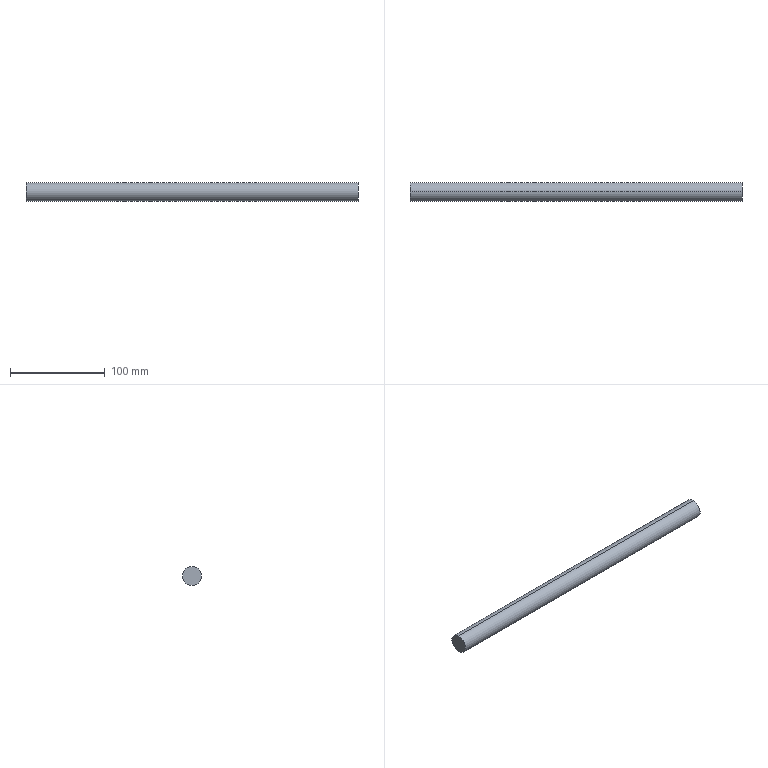Component | SolidWorks | ST60-11-2 | 1 solid | 4 faces | box 350 x 20 x 20 mm | volume 109956 mm3 | cylinder 2 | plane 2 | commonest cylinder face diameters 20 x2
build123d program:
from build123d import *

# Parameters (mm, degrees)
SKETCH1_R           = 10
BOSS_EXTRUDE1_DEPTH = 350


with BuildPart() as part:
    # Sketch1 → Boss-Extrude1 (new body)
    with BuildSketch(Plane.XY):
        Circle(SKETCH1_R)
    extrude(amount=BOSS_EXTRUDE1_DEPTH)


solid = part.part

# Placed as in the assembly
solid = solid.moved(Location((151.993, 610.454, -2151.4), (0, 90, 0)))
STEP:
#1=COLOUR_RGB('',0.7922,0.8196,0.9333);
#2=FILL_AREA_STYLE_COLOUR('',#1);
#3=FILL_AREA_STYLE('',(#2));
#4=SURFACE_STYLE_FILL_AREA(#3);
#5=SURFACE_SIDE_STYLE('',(#4));
#6=SURFACE_STYLE_USAGE(.BOTH.,#5);
#7=PRESENTATION_STYLE_ASSIGNMENT((#6));
#8=CARTESIAN_POINT('',(5.984,24.034,-84.307));
#9=VERTEX_POINT('',#8);
#10=CARTESIAN_POINT('',(5.984,24.034,-85.094));
#11=VERTEX_POINT('',#10);
#12=CARTESIAN_POINT('',(5.984,24.034,-84.701));
#13=DIRECTION('',(-1.,-0.,0.));
#14=DIRECTION('',(0.,0.,1.));
#15=AXIS2_PLACEMENT_3D('',#12,#13,#14);
#16=CIRCLE('',#15,0.3937);
#17=EDGE_CURVE('',#9,#11,#16,.T.);
#18=ORIENTED_EDGE('',*,*,#17,.F.);
#19=CARTESIAN_POINT('',(19.764,24.034,-84.307));
#20=VERTEX_POINT('',#19);
#21=CARTESIAN_POINT('',(5.984,24.034,-84.307));
#22=DIRECTION('',(1.,0.,-0.));
#23=VECTOR('',#22,39.37);
#24=LINE('',#21,#23);
#25=EDGE_CURVE('',#9,#20,#24,.T.);
#26=ORIENTED_EDGE('',*,*,#25,.T.);
#27=CARTESIAN_POINT('',(19.764,24.034,-85.094));
#28=VERTEX_POINT('',#27);
#29=CARTESIAN_POINT('',(19.764,24.034,-84.701));
#30=DIRECTION('',(-1.,-0.,0.));
#31=DIRECTION('',(0.,0.,1.));
#32=AXIS2_PLACEMENT_3D('',#29,#30,#31);
#33=CIRCLE('',#32,0.3937);
#34=EDGE_CURVE('',#20,#28,#33,.T.);
#35=ORIENTED_EDGE('',*,*,#34,.T.);
#36=CARTESIAN_POINT('',(5.984,24.034,-85.094));
#37=DIRECTION('',(1.,0.,-0.));
#38=VECTOR('',#37,39.37);
#39=LINE('',#36,#38);
#40=EDGE_CURVE('',#11,#28,#39,.T.);
#41=ORIENTED_EDGE('',*,*,#40,.F.);
#42=EDGE_LOOP('',(#18,#26,#35,#41));
#43=FACE_OUTER_BOUND('',#42,.T.);
#44=CARTESIAN_POINT('',(5.984,24.034,-84.701));
#45=DIRECTION('',(1.,0.,-0.));
#46=DIRECTION('',(0.,0.,-1.));
#47=AXIS2_PLACEMENT_3D('',#44,#45,#46);
#48=CYLINDRICAL_SURFACE('',#47,0.3937);
#49=ADVANCED_FACE('',(#43),#48,.T.);
#50=ORIENTED_EDGE('',*,*,#25,.F.);
#51=CARTESIAN_POINT('',(5.984,24.034,-84.701));
#52=DIRECTION('',(-1.,-0.,0.));
#53=DIRECTION('',(0.,0.,1.));
#54=AXIS2_PLACEMENT_3D('',#51,#52,#53);
#55=CIRCLE('',#54,0.3937);
#56=EDGE_CURVE('',#11,#9,#55,.T.);
#57=ORIENTED_EDGE('',*,*,#56,.F.);
#58=ORIENTED_EDGE('',*,*,#40,.T.);
#59=CARTESIAN_POINT('',(19.764,24.034,-84.701));
#60=DIRECTION('',(-1.,-0.,0.));
#61=DIRECTION('',(0.,0.,1.));
#62=AXIS2_PLACEMENT_3D('',#59,#60,#61);
#63=CIRCLE('',#62,0.3937);
#64=EDGE_CURVE('',#28,#20,#63,.T.);
#65=ORIENTED_EDGE('',*,*,#64,.T.);
#66=EDGE_LOOP('',(#50,#57,#58,#65));
#67=FACE_OUTER_BOUND('',#66,.T.);
#68=CARTESIAN_POINT('',(5.984,24.034,-84.701));
#69=DIRECTION('',(1.,0.,-0.));
#70=DIRECTION('',(0.,0.,-1.));
#71=AXIS2_PLACEMENT_3D('',#68,#69,#70);
#72=CYLINDRICAL_SURFACE('',#71,0.3937);
#73=ADVANCED_FACE('',(#67),#72,.T.);
#74=ORIENTED_EDGE('',*,*,#56,.T.);
#75=ORIENTED_EDGE('',*,*,#17,.T.);
#76=EDGE_LOOP('',(#74,#75));
#77=FACE_OUTER_BOUND('',#76,.T.);
#78=CARTESIAN_POINT('',(5.984,24.034,-84.701));
#79=DIRECTION('',(-1.,-0.,0.));
#80=DIRECTION('',(0.,-0.,1.));
#81=AXIS2_PLACEMENT_3D('',#78,#79,#80);
#82=PLANE('',#81);
#83=ADVANCED_FACE('',(#77),#82,.T.);
#84=ORIENTED_EDGE('',*,*,#64,.F.);
#85=ORIENTED_EDGE('',*,*,#34,.F.);
#86=EDGE_LOOP('',(#84,#85));
#87=FACE_OUTER_BOUND('',#86,.T.);
#88=CARTESIAN_POINT('',(19.764,24.034,-84.701));
#89=DIRECTION('',(-1.,-0.,0.));
#90=DIRECTION('',(0.,-0.,1.));
#91=AXIS2_PLACEMENT_3D('',#88,#89,#90);
#92=PLANE('',#91);
#93=ADVANCED_FACE('',(#87),#92,.F.);
#94=CLOSED_SHELL('',(#49,#73,#83,#93));
#95=MANIFOLD_SOLID_BREP('',#94);
#96=STYLED_ITEM('',(#7),#95);
#97=(LENGTH_UNIT()NAMED_UNIT(*)SI_UNIT($,.METRE.));
#98=LENGTH_MEASURE_WITH_UNIT(LENGTH_MEASURE(0.0254),#97);
#99=DIMENSIONAL_EXPONENTS(1.,0.,0.,0.,0.,0.,0.);
#100=(CONVERSION_BASED_UNIT('',#98)LENGTH_UNIT()NAMED_UNIT(#99));
#101=UNCERTAINTY_MEASURE_WITH_UNIT(LENGTH_MEASURE(0.00001),#100,'','');
#102=(NAMED_UNIT(*)PLANE_ANGLE_UNIT()SI_UNIT($,.RADIAN.));
#103=(NAMED_UNIT(*)SI_UNIT($,.STERADIAN.)SOLID_ANGLE_UNIT());
#104=(GEOMETRIC_REPRESENTATION_CONTEXT(3)GLOBAL_UNCERTAINTY_ASSIGNED_CONTEXT((#101))GLOBAL_UNIT_ASSIGNED_CONTEXT((#100,#102,#103))REPRESENTATION_CONTEXT('',''));
#105=MECHANICAL_DESIGN_GEOMETRIC_PRESENTATION_REPRESENTATION('',(#96),#104);
#106=PRESENTATION_LAYER_ASSIGNMENT('','',(#96));
#107=CARTESIAN_POINT('',(0.,0.,0.));
#108=DIRECTION('',(0.,0.,1.));
#109=DIRECTION('',(1.,0.,0.));
#110=AXIS2_PLACEMENT_3D('',#107,#108,#109);
#111=(LENGTH_UNIT()NAMED_UNIT(*)SI_UNIT($,.METRE.));
#112=LENGTH_MEASURE_WITH_UNIT(LENGTH_MEASURE(0.0254),#111);
#113=DIMENSIONAL_EXPONENTS(1.,0.,0.,0.,0.,0.,0.);
#114=(CONVERSION_BASED_UNIT('',#112)LENGTH_UNIT()NAMED_UNIT(#113));
#115=UNCERTAINTY_MEASURE_WITH_UNIT(LENGTH_MEASURE(0.00001),#114,'','');
#116=(NAMED_UNIT(*)PLANE_ANGLE_UNIT()SI_UNIT($,.RADIAN.));
#117=(NAMED_UNIT(*)SI_UNIT($,.STERADIAN.)SOLID_ANGLE_UNIT());
#118=(GEOMETRIC_REPRESENTATION_CONTEXT(3)GLOBAL_UNCERTAINTY_ASSIGNED_CONTEXT((#115))GLOBAL_UNIT_ASSIGNED_CONTEXT((#114,#116,#117))REPRESENTATION_CONTEXT('',''));
#119=ADVANCED_BREP_SHAPE_REPRESENTATION('',(#95,#110),#118);